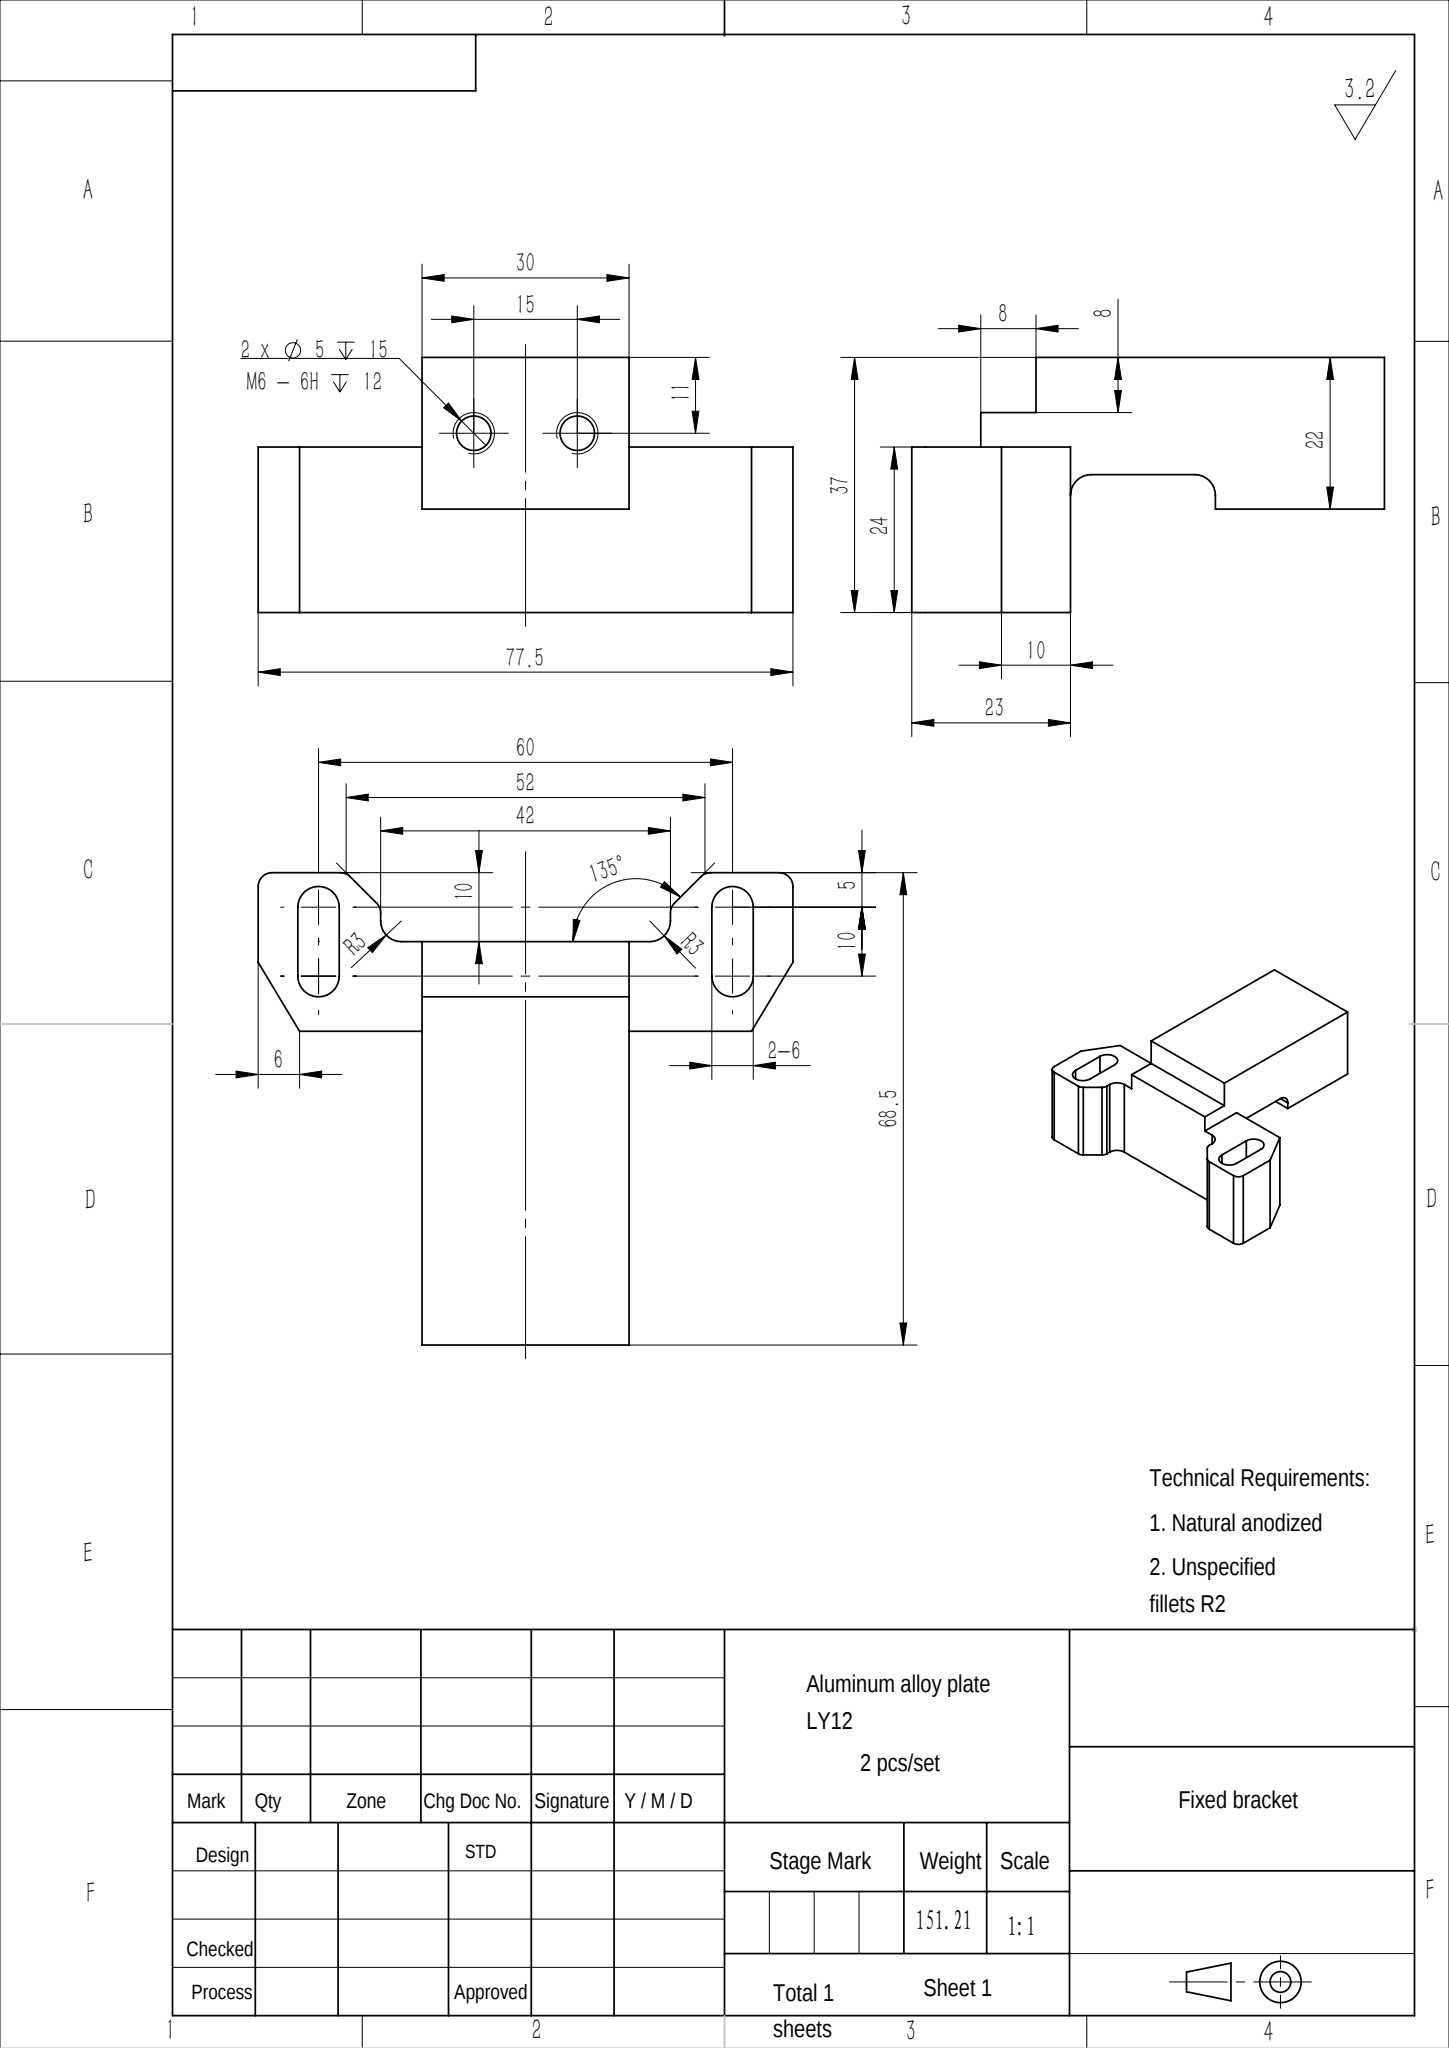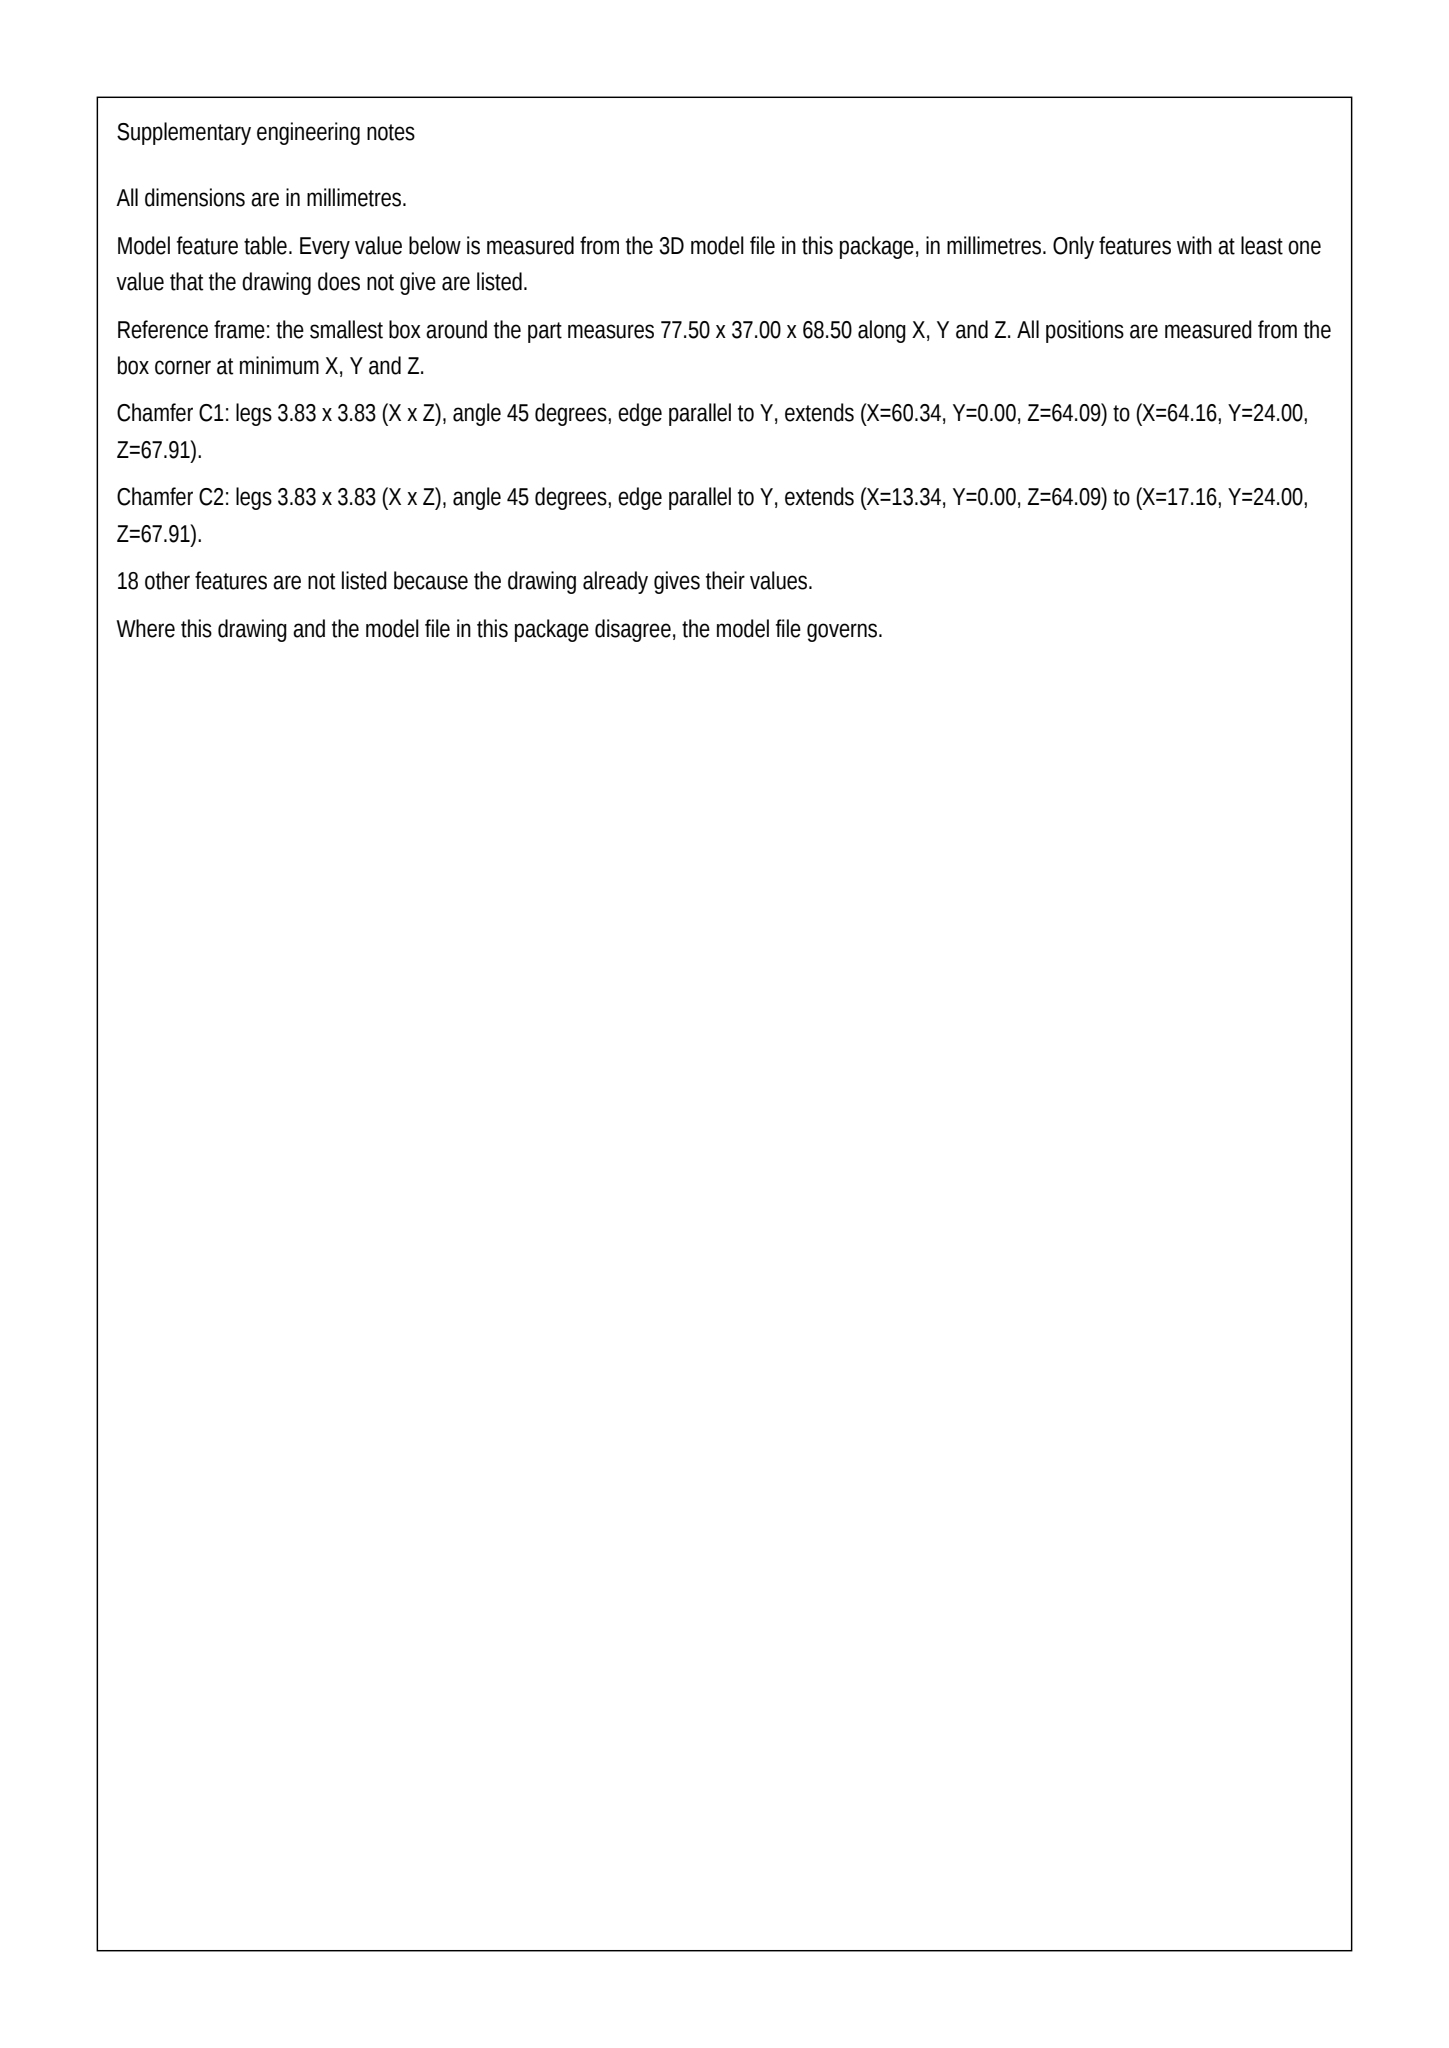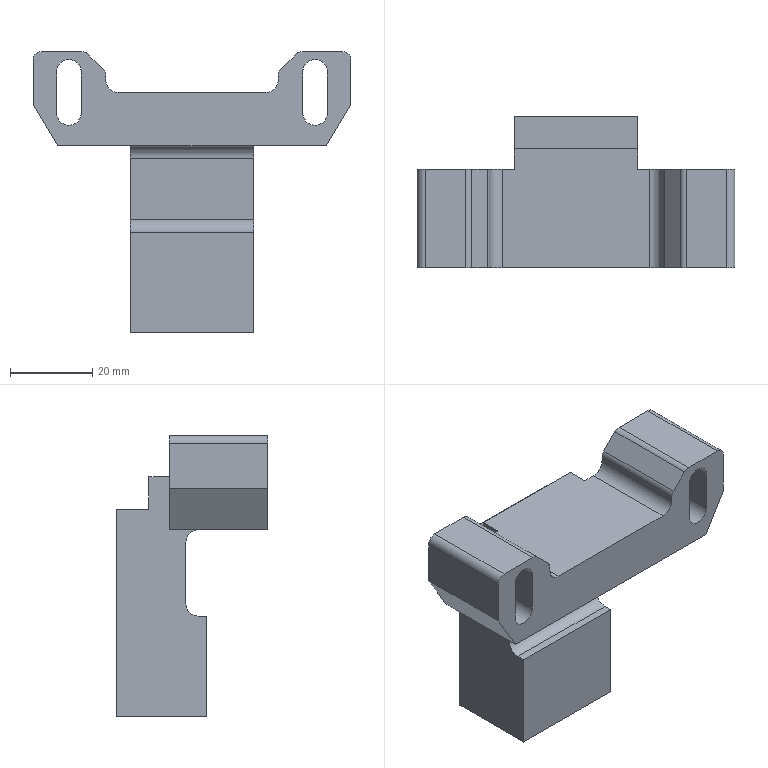Part | SolidWorks | mm | material Aluminum alloy plate LY12 | 1 solid | 52 faces | box 77.5 x 37 x 68.5 mm | volume 56003 mm3 | plane 28 | cylinder 20 | cone 4 | commonest cylinder face diameters 6 x10 4 x6 5 x4
build123d program:
from build123d import *

# Parameters (mm, degrees)
SKETCH1_W             = 30
SKETCH1_H             = 68.5
BOSS_EXTRUDE1_DEPTH   = 22
BOSS_EXTRUDE2_START   = -13
SKETCH2_W             = 77.5
SKETCH2_H             = 23
BOSS_EXTRUDE2_DEPTH   = 24
SKETCH4_W             = 42
SKETCH4_H             = 10
CUT_EXTRUDE2_DEPTH    = 87.964
CUT_EXTRUDE3_DEPTH    = 83.279
M6_TAPPED_HOLE1_D     = 5
M6_TAPPED_HOLE1_DEPTH = 15
M6_TAPPED_HOLE1_TIP   = 1.502
FILLET1_R             = 3
CHAMFER2_SIZE         = 5
FILLET3_R             = 2
CHAMFER3_SIZE         = 6
CHAMFER3_SIZE2        = 10
CHAMFER4_SIZE         = 10
CHAMFER4_SIZE2        = 6
SKETCH10_W            = 8
SKETCH10_H            = 8
CUT_EXTRUDE5_DEPTH    = 90.807
SKETCH11_W            = 21
SKETCH11_H            = 5
CUT_EXTRUDE6_DEPTH    = 90.807
FILLET4_R             = 3


with BuildPart() as part:
    # Sketch1 → Boss-Extrude1 (new body)
    with BuildSketch(Plane(origin=(0, 0, 0), x_dir=(1, 0, 0), z_dir=(0, 1, 0))):
        with Locations((0, 34.25)):
            Rectangle(SKETCH1_W, SKETCH1_H)
    extrude(amount=BOSS_EXTRUDE1_DEPTH)

    # Sketch2 → Boss-Extrude2 (add)
    with BuildSketch(Plane(origin=(0, 22, 0), x_dir=(1, 0, 0), z_dir=(0, 1, 0)).offset(BOSS_EXTRUDE2_START)):
        with Locations((0, 11.5)):
            Rectangle(SKETCH2_W, SKETCH2_H)
    extrude(amount=-BOSS_EXTRUDE2_DEPTH)

    # Sketch4 → Cut-Extrude2 (cut, through all)
    with BuildSketch(Plane(origin=(0, 22, 0), x_dir=(1, 0, 0), z_dir=(0, 1, 0))):
        with Locations((0, 5)):
            Rectangle(SKETCH4_W, SKETCH4_H)
    extrude(amount=-CUT_EXTRUDE2_DEPTH, mode=Mode.SUBTRACT)

    # Sketch5 → Cut-Extrude3 (cut, through all)
    with BuildSketch(Plane(origin=(0, 9, 0), x_dir=(1, 0, 0), z_dir=(0, 1, 0))):
        with BuildLine():
            Line((-27, 15), (-27, 5))
            ThreePointArc((-27, 5), (-30, 2), (-33, 5))
            Line((-33, 5), (-33, 15))
            ThreePointArc((-33, 15), (-30, 18), (-27, 15))
        make_face()
        with BuildLine():
            Line((27, 15), (27, 5))
            ThreePointArc((27, 5), (30, 2), (33, 5))
            Line((33, 5), (33, 15))
            ThreePointArc((33, 15), (30, 18), (27, 15))
        make_face()
    extrude(amount=-CUT_EXTRUDE3_DEPTH, mode=Mode.SUBTRACT)

    # M6 Tapped Hole1
    with Locations(Plane(origin=(0, 0, -68.5), x_dir=(-1, 0, 0), z_dir=(0, 0, -1))):
        with Locations((7.5, 11), (-7.5, 11)):
            Hole(M6_TAPPED_HOLE1_D / 2, depth=M6_TAPPED_HOLE1_DEPTH)
            with Locations((0, 0, -(M6_TAPPED_HOLE1_DEPTH + M6_TAPPED_HOLE1_TIP / 2))):  # 118° drill point
                Cone(0, M6_TAPPED_HOLE1_D / 2, M6_TAPPED_HOLE1_TIP, mode=Mode.SUBTRACT)

    # Fillet1
    fillet1_edges = [part.edges().sort_by_distance(p)[0] for p in [
        (-21, -3, -10),
        (21, -3, -10),
    ]]
    fillet(fillet1_edges, radius=FILLET1_R)

    # Chamfer2
    chamfer2_edges = [part.edges().sort_by_distance(p)[0] for p in [
        (-21, -3, 0),
        (21, -3, 0),
    ]]
    chamfer(chamfer2_edges, length=CHAMFER2_SIZE)

    # Fillet3
    fillet3_edges = [part.edges().sort_by_distance(p)[0] for p in [
        (21, -3, -5),
        (26, -3, 0),
        (-26, -3, 0),
        (-21, -3, -5),
        (38.75, -3, 0),
        (-38.75, -3, 0),
    ]]
    fillet(fillet3_edges, radius=FILLET3_R)

    # Chamfer3
    chamfer3_edges = [part.edges().sort_by_distance(p)[0] for p in [
        (38.75, -3, -23),
    ]]
    chamfer3_side = [part.faces().sort_by_distance(p)[0] for p in [
        (0, -4.274, -23),
    ]]
    chamfer(chamfer3_edges, length=CHAMFER3_SIZE, length2=CHAMFER3_SIZE2, reference=chamfer3_side[0])

    # Chamfer4
    chamfer4_edges = [part.edges().sort_by_distance(p)[0] for p in [
        (-38.75, -3, -23),
    ]]
    chamfer4_side = [part.faces().sort_by_distance(p)[0] for p in [
        (-38.75, -3, -12.5),
    ]]
    chamfer(chamfer4_edges, length=CHAMFER4_SIZE, length2=CHAMFER4_SIZE2, reference=chamfer4_side[0])

    # Sketch10 → Cut-Extrude5 (cut, through all)
    with BuildSketch(Plane.ZY.offset(15)):
        with Locations((-14, 18)):
            Rectangle(SKETCH10_W, SKETCH10_H)
    extrude(amount=-CUT_EXTRUDE5_DEPTH, mode=Mode.SUBTRACT)

    # Sketch11 → Cut-Extrude6 (cut, through all)
    with BuildSketch(Plane.ZY.offset(15)):
        with Locations((-33.5, 2.5)):
            Rectangle(SKETCH11_W, SKETCH11_H)
    extrude(amount=-CUT_EXTRUDE6_DEPTH, mode=Mode.SUBTRACT)

    # Fillet4
    fillet4_edges = [part.edges().sort_by_distance(p)[0] for p in [
        (0, 5, -44),
        (0, 5, -23),
    ]]
    fillet(fillet4_edges, radius=FILLET4_R)


solid = part.part